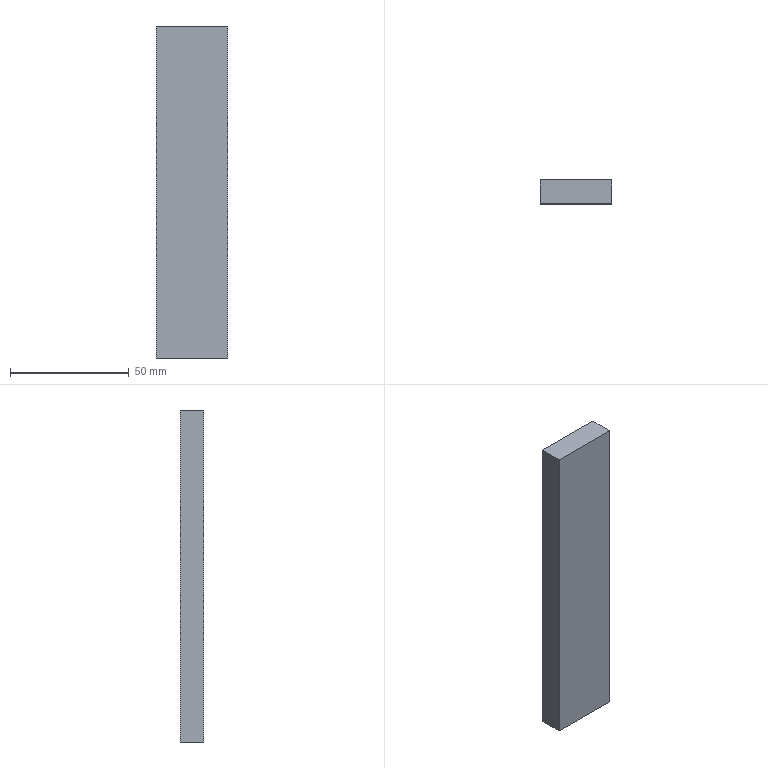Component | SolidWorks | Shim-7 | 1 solid | 6 faces | box 30 x 10 x 140 mm | volume 42000 mm3 | plane 6
build123d program:
from build123d import *

# Parameters (mm, degrees)
SKETCH2_W           = 30
SKETCH2_H           = 140
BOSS_EXTRUDE1_DEPTH = 10


with BuildPart() as part:
    # Sketch2 → Boss-Extrude1 (new body)
    with BuildSketch(Plane.XY):
        with Locations((-290.265, 14.821)):
            Rectangle(SKETCH2_W, SKETCH2_H)
    extrude(amount=BOSS_EXTRUDE1_DEPTH)


solid = part.part

# Placed as in the assembly
solid = solid.moved(Location((62.265, 160, -28.821), (90, 0, 0)))
STEP:
#1=COLOUR_RGB('',0.7922,0.8196,0.9333);
#2=FILL_AREA_STYLE_COLOUR('',#1);
#3=FILL_AREA_STYLE('',(#2));
#4=SURFACE_STYLE_FILL_AREA(#3);
#5=SURFACE_SIDE_STYLE('',(#4));
#6=SURFACE_STYLE_USAGE(.BOTH.,#5);
#7=PRESENTATION_STYLE_ASSIGNMENT((#6));
#8=CARTESIAN_POINT('',(-9.567,5.906,-3.307));
#9=VERTEX_POINT('',#8);
#10=CARTESIAN_POINT('',(-9.567,5.906,2.205));
#11=VERTEX_POINT('',#10);
#12=CARTESIAN_POINT('',(-9.567,5.906,-3.307));
#13=DIRECTION('',(0.,0.,1.));
#14=VECTOR('',#13,39.37);
#15=LINE('',#12,#14);
#16=EDGE_CURVE('',#9,#11,#15,.T.);
#17=ORIENTED_EDGE('',*,*,#16,.T.);
#18=CARTESIAN_POINT('',(-9.567,6.299,2.205));
#19=VERTEX_POINT('',#18);
#20=CARTESIAN_POINT('',(-9.567,6.299,2.205));
#21=DIRECTION('',(0.,-1.,0.));
#22=VECTOR('',#21,39.37);
#23=LINE('',#20,#22);
#24=EDGE_CURVE('',#19,#11,#23,.T.);
#25=ORIENTED_EDGE('',*,*,#24,.F.);
#26=CARTESIAN_POINT('',(-9.567,6.299,-3.307));
#27=VERTEX_POINT('',#26);
#28=CARTESIAN_POINT('',(-9.567,6.299,-3.307));
#29=DIRECTION('',(0.,0.,1.));
#30=VECTOR('',#29,39.37);
#31=LINE('',#28,#30);
#32=EDGE_CURVE('',#27,#19,#31,.T.);
#33=ORIENTED_EDGE('',*,*,#32,.F.);
#34=CARTESIAN_POINT('',(-9.567,6.299,-3.307));
#35=DIRECTION('',(0.,-1.,0.));
#36=VECTOR('',#35,39.37);
#37=LINE('',#34,#36);
#38=EDGE_CURVE('',#27,#9,#37,.T.);
#39=ORIENTED_EDGE('',*,*,#38,.T.);
#40=EDGE_LOOP('',(#17,#25,#33,#39));
#41=FACE_OUTER_BOUND('',#40,.T.);
#42=CARTESIAN_POINT('',(-9.567,6.299,-3.307));
#43=DIRECTION('',(1.,0.,0.));
#44=DIRECTION('',(0.,-1.,0.));
#45=AXIS2_PLACEMENT_3D('',#42,#43,#44);
#46=PLANE('',#45);
#47=ADVANCED_FACE('',(#41),#46,.F.);
#48=CARTESIAN_POINT('',(-8.386,5.906,2.205));
#49=VERTEX_POINT('',#48);
#50=CARTESIAN_POINT('',(-9.567,5.906,2.205));
#51=DIRECTION('',(1.,0.,0.));
#52=VECTOR('',#51,39.37);
#53=LINE('',#50,#52);
#54=EDGE_CURVE('',#11,#49,#53,.T.);
#55=ORIENTED_EDGE('',*,*,#54,.T.);
#56=CARTESIAN_POINT('',(-8.386,6.299,2.205));
#57=VERTEX_POINT('',#56);
#58=CARTESIAN_POINT('',(-8.386,6.299,2.205));
#59=DIRECTION('',(0.,-1.,0.));
#60=VECTOR('',#59,39.37);
#61=LINE('',#58,#60);
#62=EDGE_CURVE('',#57,#49,#61,.T.);
#63=ORIENTED_EDGE('',*,*,#62,.F.);
#64=CARTESIAN_POINT('',(-9.567,6.299,2.205));
#65=DIRECTION('',(1.,0.,0.));
#66=VECTOR('',#65,39.37);
#67=LINE('',#64,#66);
#68=EDGE_CURVE('',#19,#57,#67,.T.);
#69=ORIENTED_EDGE('',*,*,#68,.F.);
#70=ORIENTED_EDGE('',*,*,#24,.T.);
#71=EDGE_LOOP('',(#55,#63,#69,#70));
#72=FACE_OUTER_BOUND('',#71,.T.);
#73=CARTESIAN_POINT('',(-9.567,6.299,2.205));
#74=DIRECTION('',(0.,0.,-1.));
#75=DIRECTION('',(0.,1.,0.));
#76=AXIS2_PLACEMENT_3D('',#73,#74,#75);
#77=PLANE('',#76);
#78=ADVANCED_FACE('',(#72),#77,.F.);
#79=CARTESIAN_POINT('',(-8.386,5.906,-3.307));
#80=VERTEX_POINT('',#79);
#81=CARTESIAN_POINT('',(-8.386,5.906,-3.307));
#82=DIRECTION('',(0.,0.,-1.));
#83=VECTOR('',#82,39.37);
#84=LINE('',#81,#83);
#85=EDGE_CURVE('',#49,#80,#84,.T.);
#86=ORIENTED_EDGE('',*,*,#85,.T.);
#87=CARTESIAN_POINT('',(-8.386,6.299,-3.307));
#88=VERTEX_POINT('',#87);
#89=CARTESIAN_POINT('',(-8.386,6.299,-3.307));
#90=DIRECTION('',(0.,-1.,0.));
#91=VECTOR('',#90,39.37);
#92=LINE('',#89,#91);
#93=EDGE_CURVE('',#88,#80,#92,.T.);
#94=ORIENTED_EDGE('',*,*,#93,.F.);
#95=CARTESIAN_POINT('',(-8.386,6.299,-3.307));
#96=DIRECTION('',(0.,0.,-1.));
#97=VECTOR('',#96,39.37);
#98=LINE('',#95,#97);
#99=EDGE_CURVE('',#57,#88,#98,.T.);
#100=ORIENTED_EDGE('',*,*,#99,.F.);
#101=ORIENTED_EDGE('',*,*,#62,.T.);
#102=EDGE_LOOP('',(#86,#94,#100,#101));
#103=FACE_OUTER_BOUND('',#102,.T.);
#104=CARTESIAN_POINT('',(-8.386,6.299,-3.307));
#105=DIRECTION('',(-1.,0.,0.));
#106=DIRECTION('',(0.,1.,0.));
#107=AXIS2_PLACEMENT_3D('',#104,#105,#106);
#108=PLANE('',#107);
#109=ADVANCED_FACE('',(#103),#108,.F.);
#110=CARTESIAN_POINT('',(-9.567,5.906,-3.307));
#111=DIRECTION('',(-1.,0.,0.));
#112=VECTOR('',#111,39.37);
#113=LINE('',#110,#112);
#114=EDGE_CURVE('',#80,#9,#113,.T.);
#115=ORIENTED_EDGE('',*,*,#114,.T.);
#116=ORIENTED_EDGE('',*,*,#38,.F.);
#117=CARTESIAN_POINT('',(-9.567,6.299,-3.307));
#118=DIRECTION('',(-1.,0.,0.));
#119=VECTOR('',#118,39.37);
#120=LINE('',#117,#119);
#121=EDGE_CURVE('',#88,#27,#120,.T.);
#122=ORIENTED_EDGE('',*,*,#121,.F.);
#123=ORIENTED_EDGE('',*,*,#93,.T.);
#124=EDGE_LOOP('',(#115,#116,#122,#123));
#125=FACE_OUTER_BOUND('',#124,.T.);
#126=CARTESIAN_POINT('',(-9.567,6.299,-3.307));
#127=DIRECTION('',(0.,0.,1.));
#128=DIRECTION('',(0.,-1.,0.));
#129=AXIS2_PLACEMENT_3D('',#126,#127,#128);
#130=PLANE('',#129);
#131=ADVANCED_FACE('',(#125),#130,.F.);
#132=ORIENTED_EDGE('',*,*,#32,.T.);
#133=ORIENTED_EDGE('',*,*,#68,.T.);
#134=ORIENTED_EDGE('',*,*,#99,.T.);
#135=ORIENTED_EDGE('',*,*,#121,.T.);
#136=EDGE_LOOP('',(#132,#133,#134,#135));
#137=FACE_OUTER_BOUND('',#136,.T.);
#138=CARTESIAN_POINT('',(2.451,6.299,0.03232));
#139=DIRECTION('',(0.,1.,0.));
#140=DIRECTION('',(1.,0.,0.));
#141=AXIS2_PLACEMENT_3D('',#138,#139,#140);
#142=PLANE('',#141);
#143=ADVANCED_FACE('',(#137),#142,.T.);
#144=ORIENTED_EDGE('',*,*,#16,.F.);
#145=ORIENTED_EDGE('',*,*,#114,.F.);
#146=ORIENTED_EDGE('',*,*,#85,.F.);
#147=ORIENTED_EDGE('',*,*,#54,.F.);
#148=EDGE_LOOP('',(#144,#145,#146,#147));
#149=FACE_OUTER_BOUND('',#148,.T.);
#150=CARTESIAN_POINT('',(2.451,5.906,0.03232));
#151=DIRECTION('',(0.,1.,0.));
#152=DIRECTION('',(1.,0.,0.));
#153=AXIS2_PLACEMENT_3D('',#150,#151,#152);
#154=PLANE('',#153);
#155=ADVANCED_FACE('',(#149),#154,.F.);
#156=CLOSED_SHELL('',(#47,#78,#109,#131,#143,#155));
#157=MANIFOLD_SOLID_BREP('',#156);
#158=STYLED_ITEM('',(#7),#157);
#159=PRESENTATION_LAYER_ASSIGNMENT('','',(#158));
#160=CARTESIAN_POINT('',(0.,0.,0.));
#161=DIRECTION('',(0.,0.,1.));
#162=DIRECTION('',(1.,0.,0.));
#163=AXIS2_PLACEMENT_3D('',#160,#161,#162);
#164=(LENGTH_UNIT()NAMED_UNIT(*)SI_UNIT($,.METRE.));
#165=LENGTH_MEASURE_WITH_UNIT(LENGTH_MEASURE(0.0254),#164);
#166=DIMENSIONAL_EXPONENTS(1.,0.,0.,0.,0.,0.,0.);
#167=(CONVERSION_BASED_UNIT('',#165)LENGTH_UNIT()NAMED_UNIT(#166));
#168=UNCERTAINTY_MEASURE_WITH_UNIT(LENGTH_MEASURE(0.00001),#167,'','');
#169=(NAMED_UNIT(*)PLANE_ANGLE_UNIT()SI_UNIT($,.RADIAN.));
#170=(NAMED_UNIT(*)SI_UNIT($,.STERADIAN.)SOLID_ANGLE_UNIT());
#171=(GEOMETRIC_REPRESENTATION_CONTEXT(3)GLOBAL_UNCERTAINTY_ASSIGNED_CONTEXT((#168))GLOBAL_UNIT_ASSIGNED_CONTEXT((#167,#169,#170))REPRESENTATION_CONTEXT('',''));
#172=ADVANCED_BREP_SHAPE_REPRESENTATION('',(#157,#163),#171);
#173=(LENGTH_UNIT()NAMED_UNIT(*)SI_UNIT($,.METRE.));
#174=LENGTH_MEASURE_WITH_UNIT(LENGTH_MEASURE(0.0254),#173);
#175=DIMENSIONAL_EXPONENTS(1.,0.,0.,0.,0.,0.,0.);
#176=(CONVERSION_BASED_UNIT('',#174)LENGTH_UNIT()NAMED_UNIT(#175));
#177=UNCERTAINTY_MEASURE_WITH_UNIT(LENGTH_MEASURE(0.00001),#176,'','');
#178=(NAMED_UNIT(*)PLANE_ANGLE_UNIT()SI_UNIT($,.RADIAN.));
#179=(NAMED_UNIT(*)SI_UNIT($,.STERADIAN.)SOLID_ANGLE_UNIT());
#180=(GEOMETRIC_REPRESENTATION_CONTEXT(3)GLOBAL_UNCERTAINTY_ASSIGNED_CONTEXT((#177))GLOBAL_UNIT_ASSIGNED_CONTEXT((#176,#178,#179))REPRESENTATION_CONTEXT('',''));
#181=MECHANICAL_DESIGN_GEOMETRIC_PRESENTATION_REPRESENTATION('',(#158),#180);